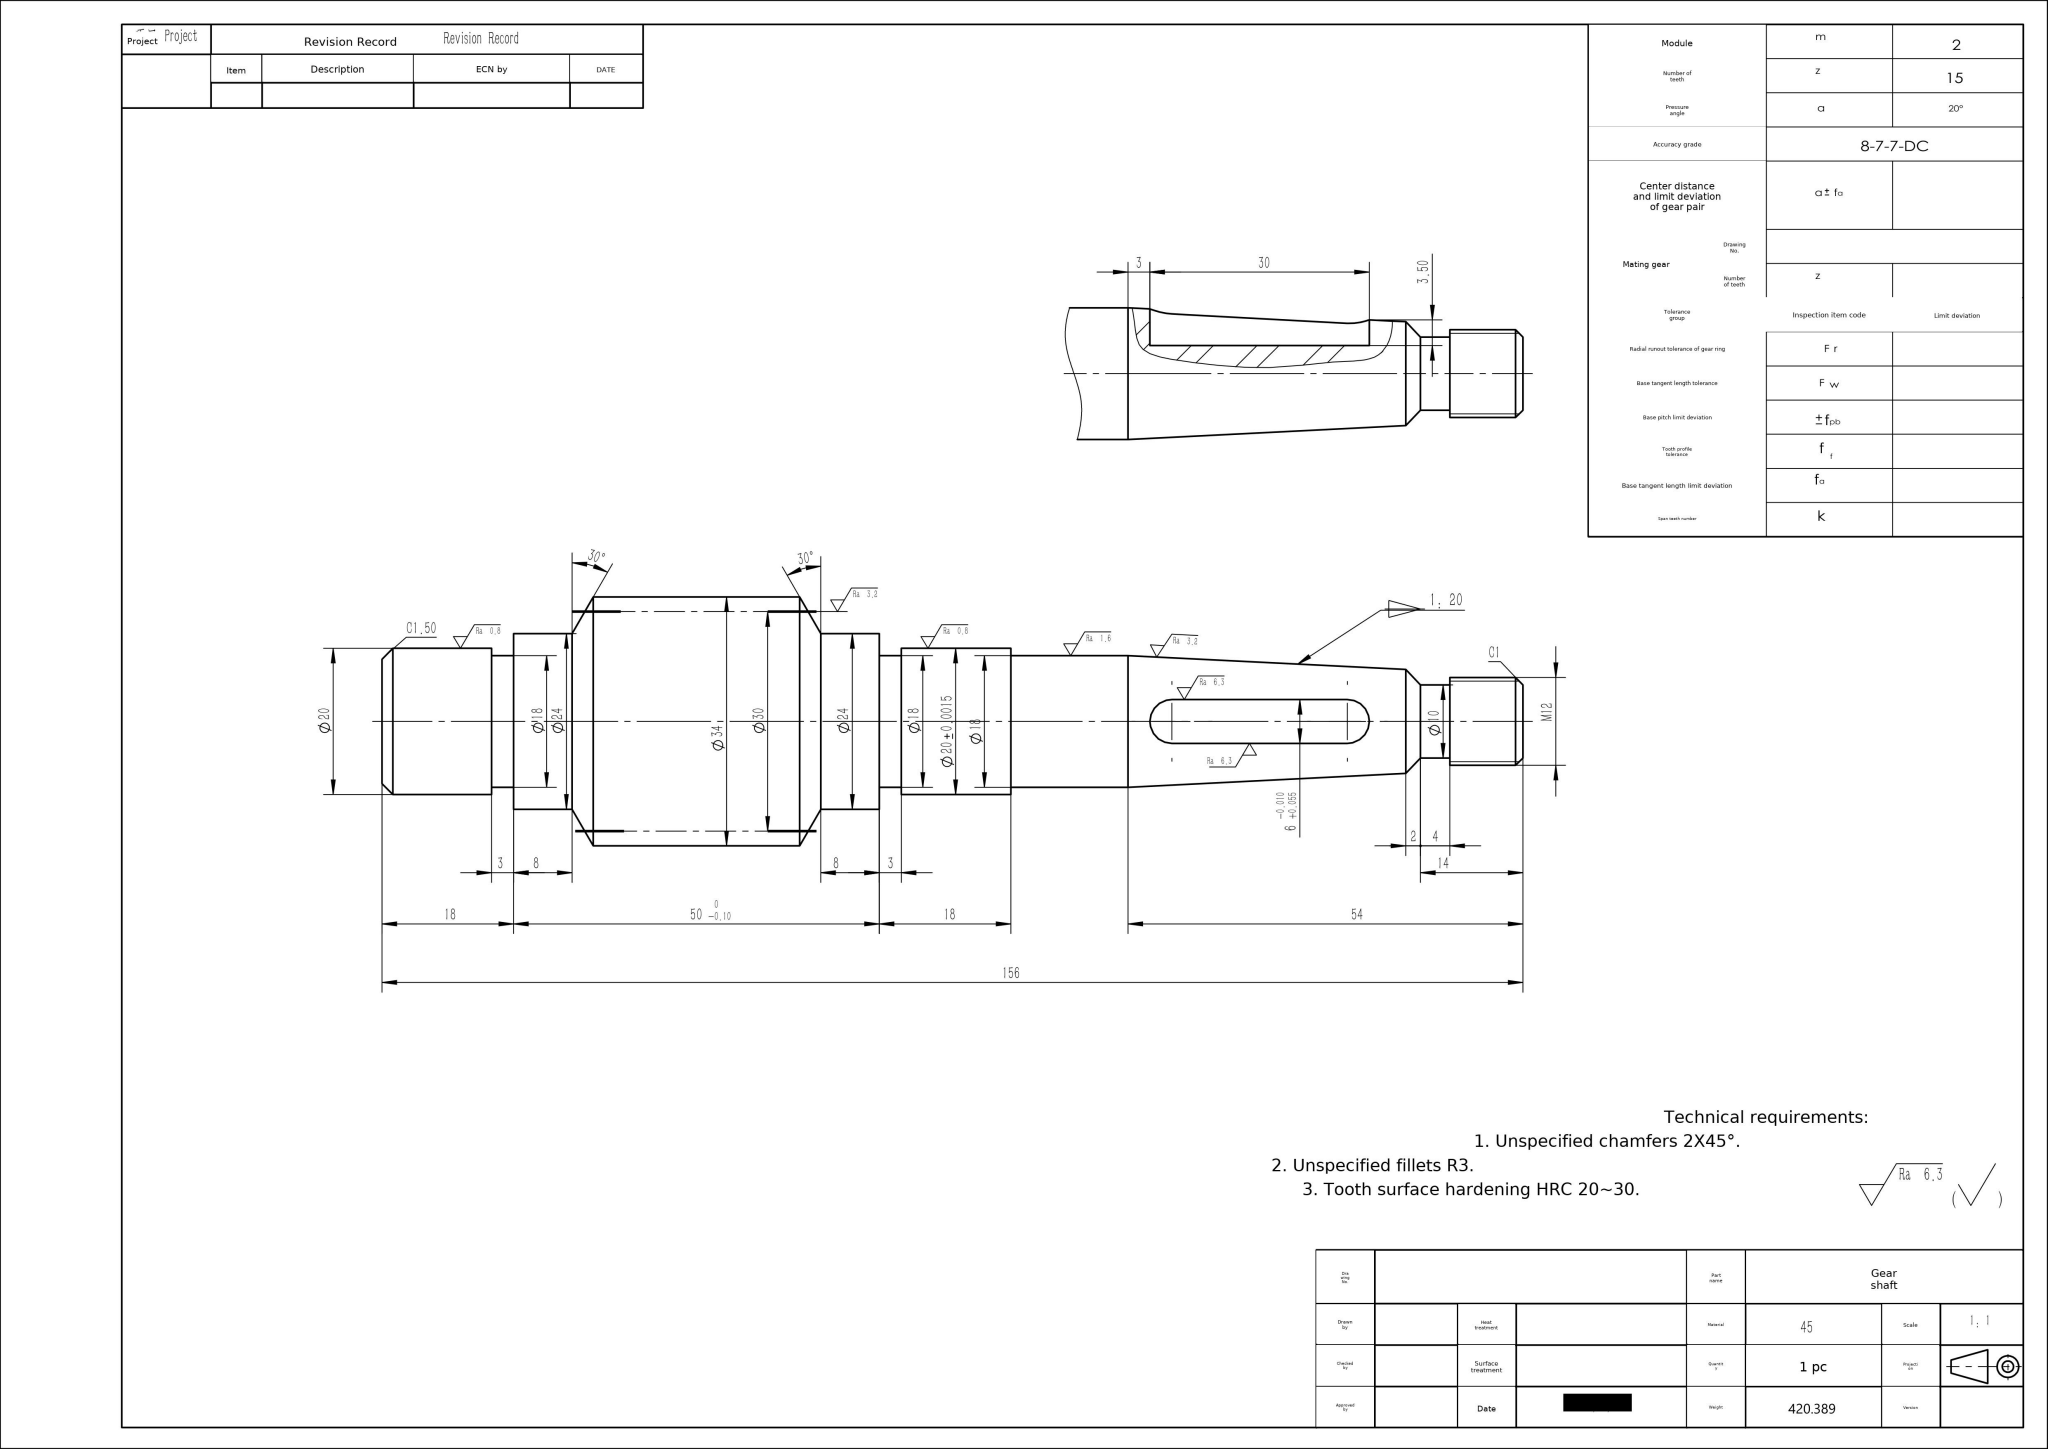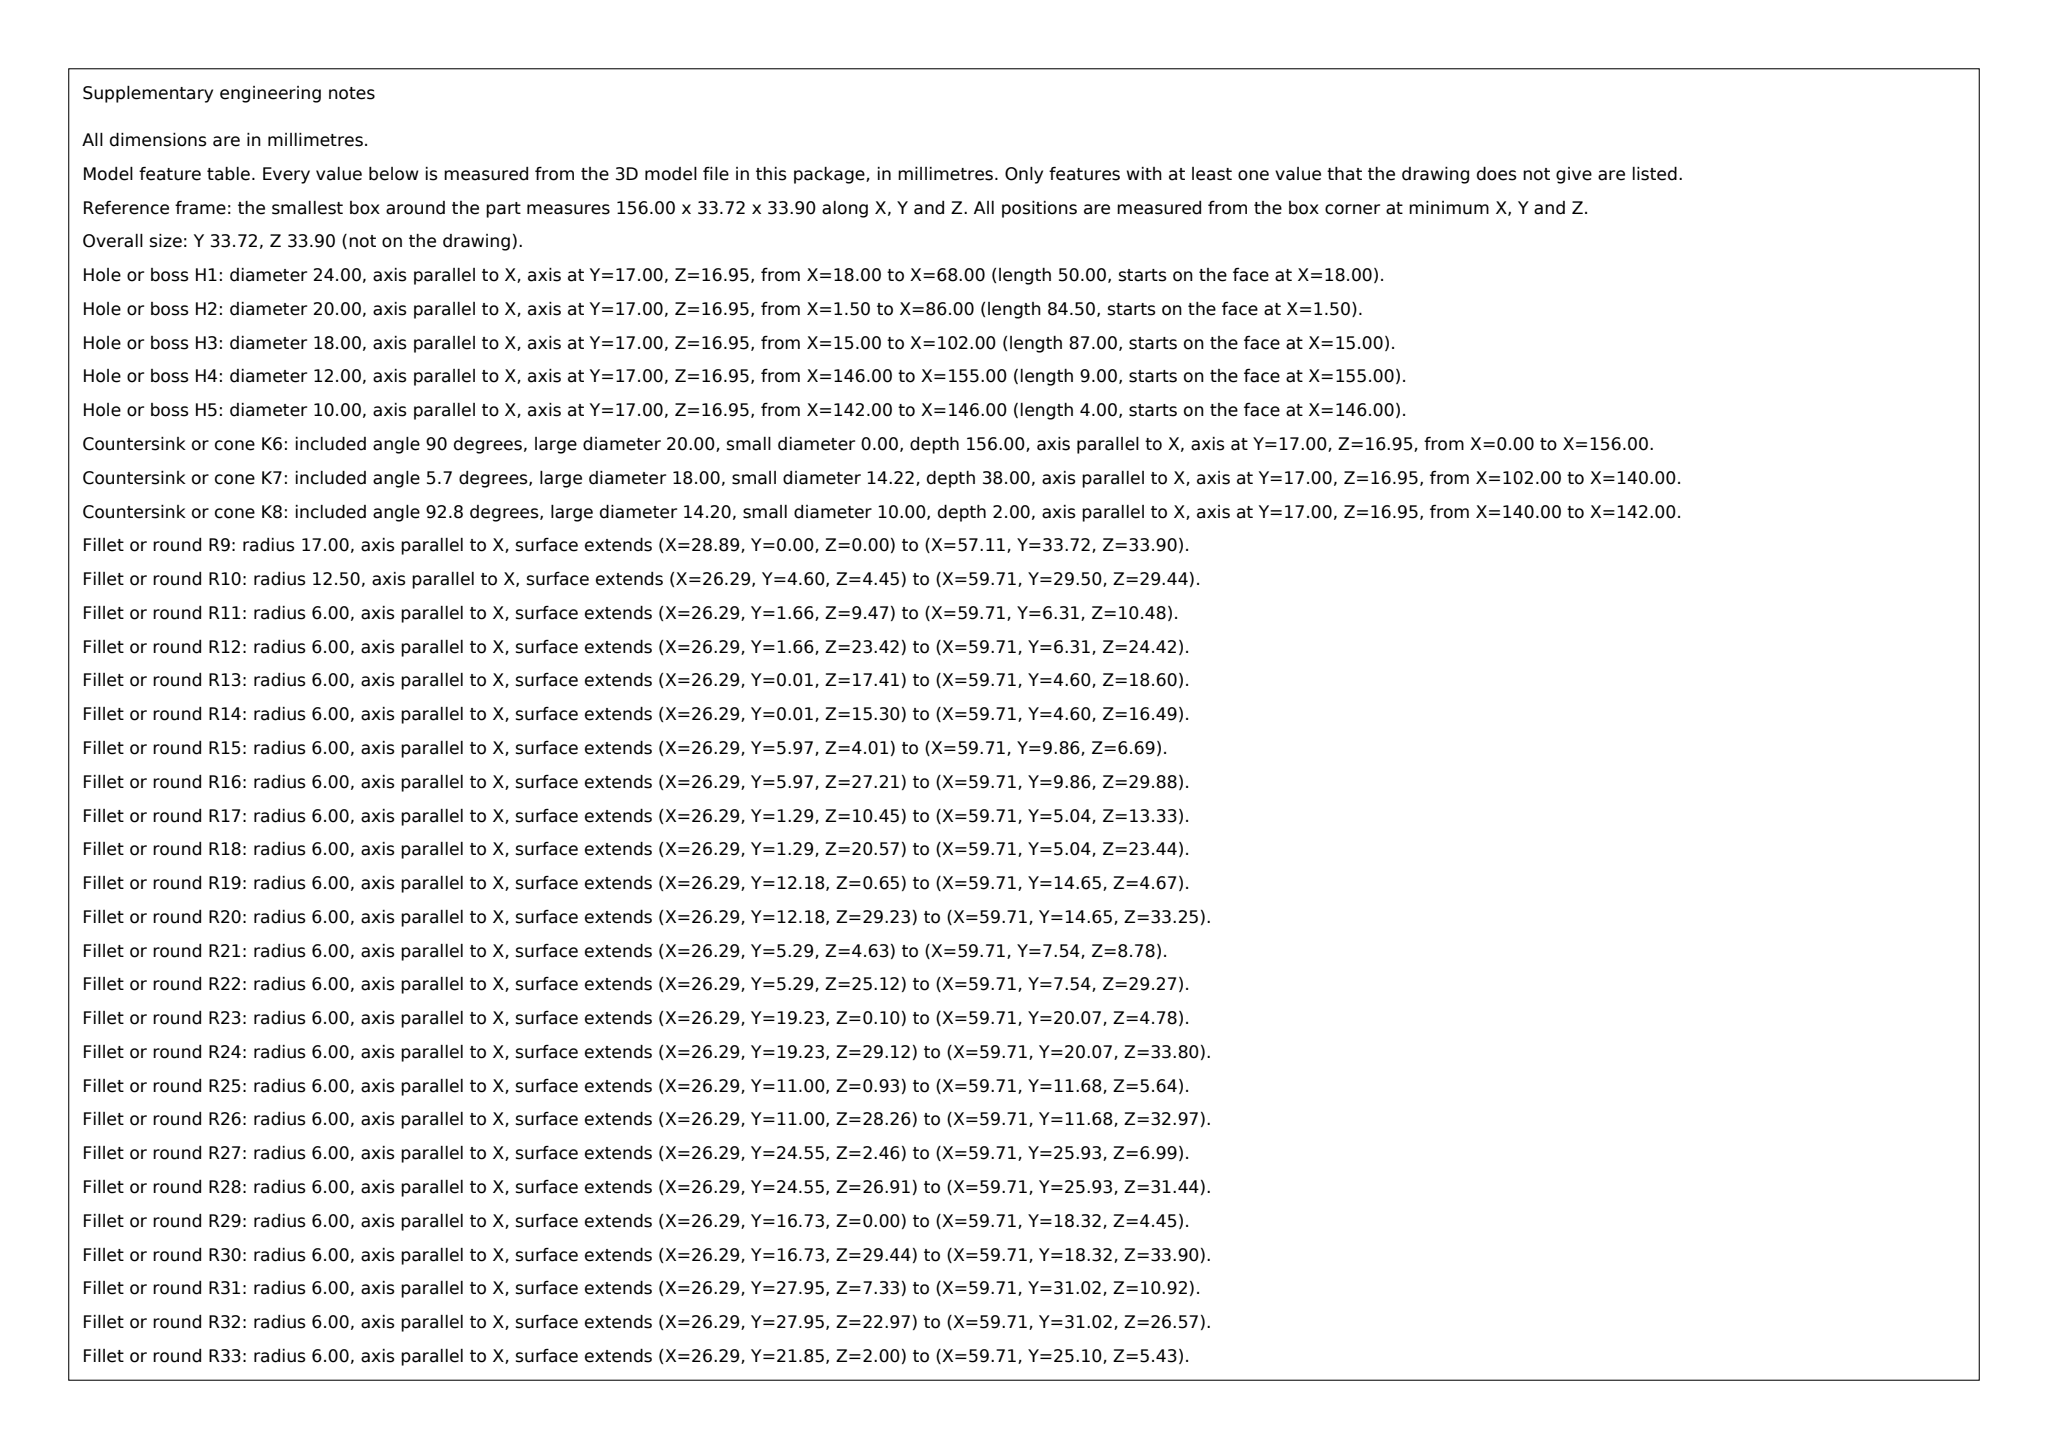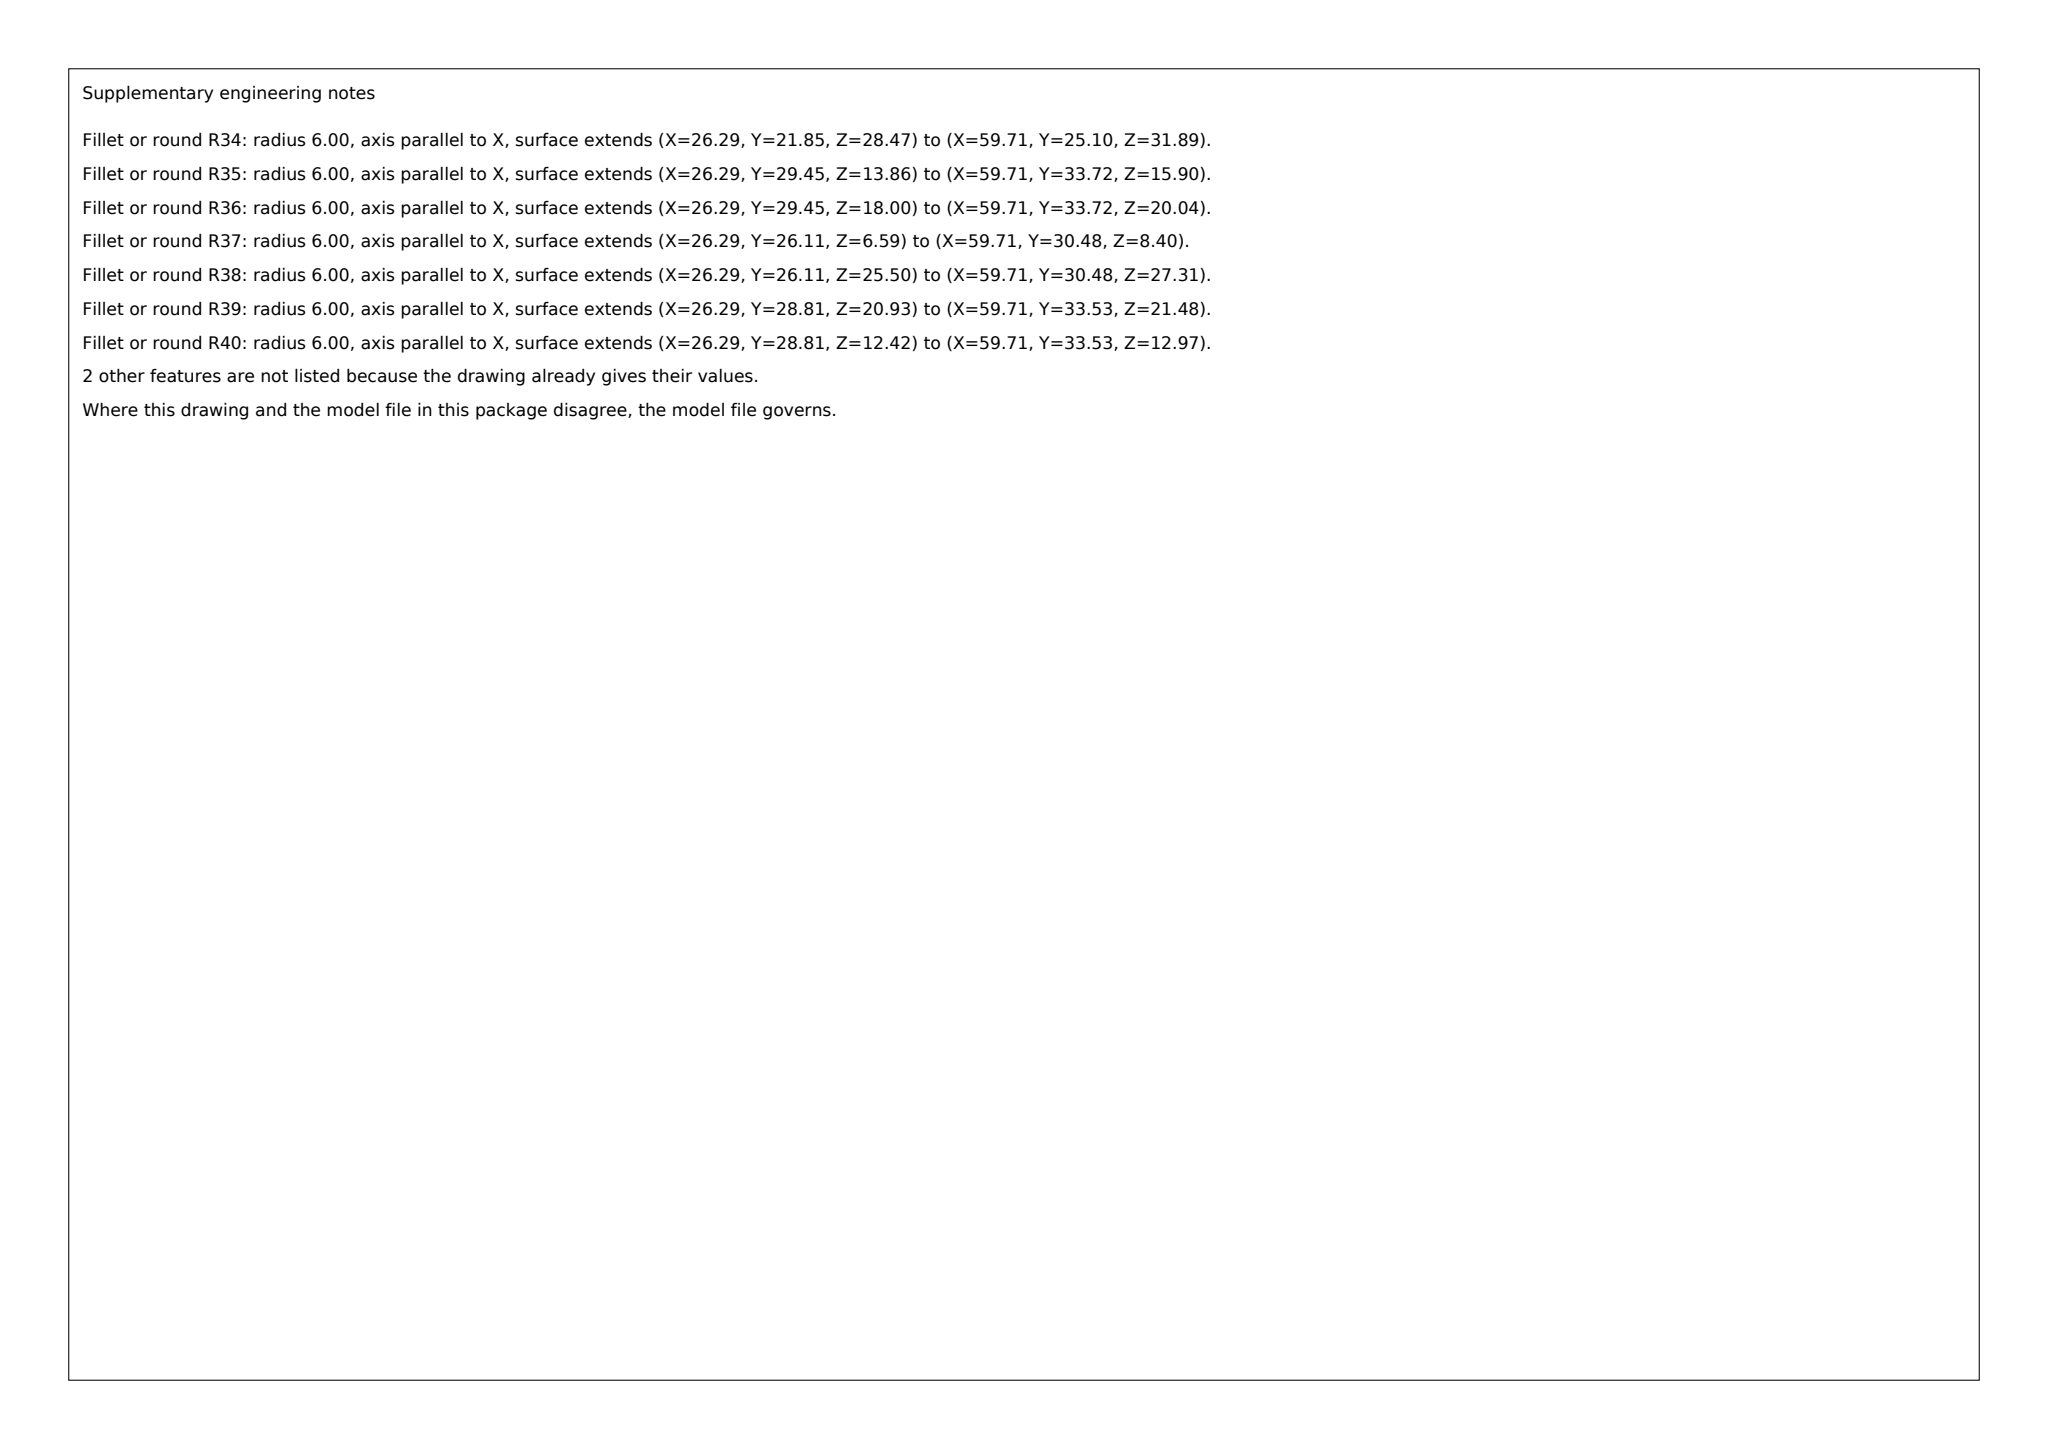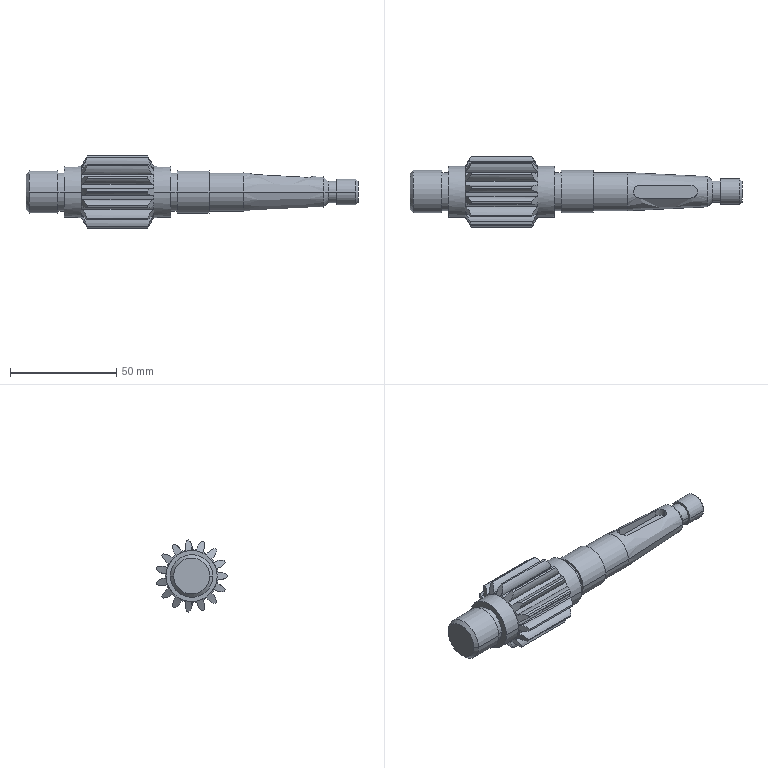Part | SolidWorks | mm | material 45 | 1 solid | 109 faces | box 156 x 33.72 x 33.9 mm | volume 53281 mm3 | cylinder 86 | cone 12 | plane 11 | commonest cylinder face diameters 12 x36 34 x15 24.998 x15 18 x6 24 x4 20 x4 6 x4 10 x2